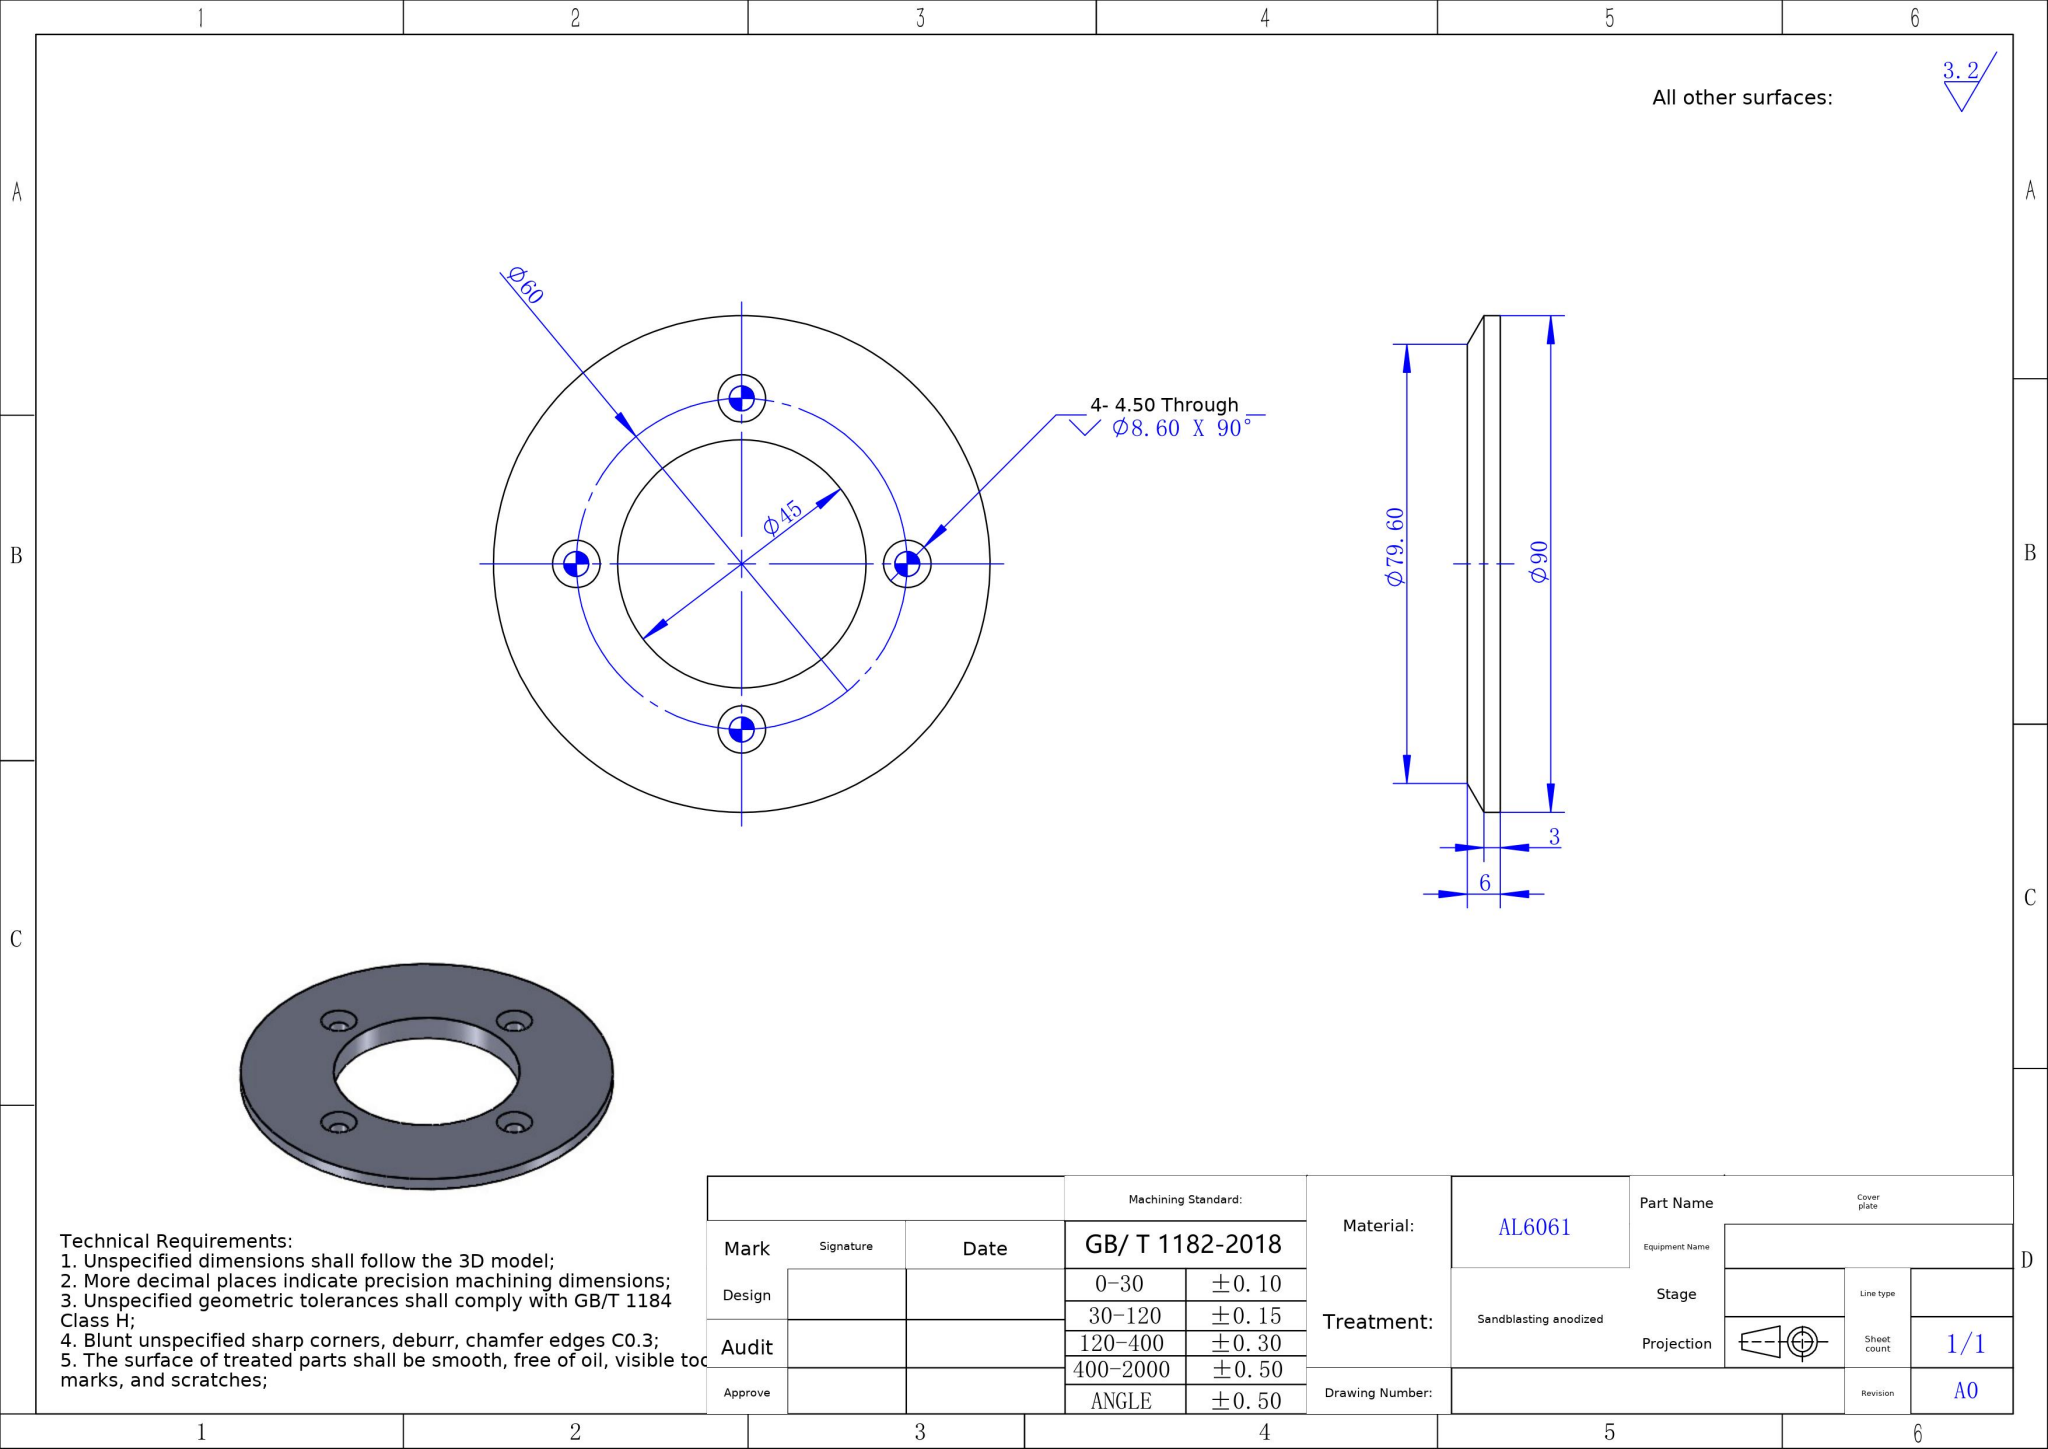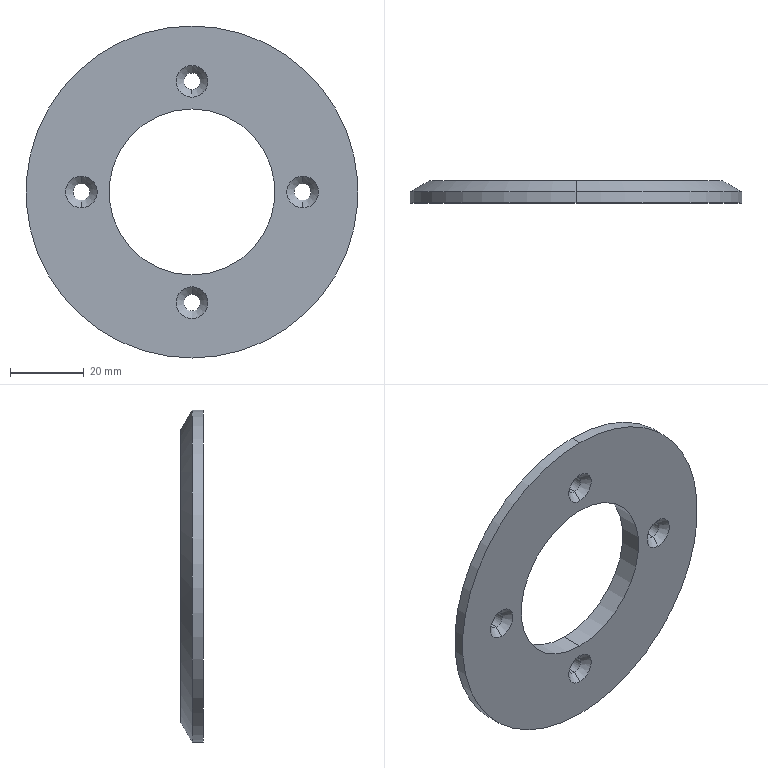Part | SolidWorks | mm | material AL6061 | 1 solid | 24 faces | box 90 x 6 x 90 mm | volume 25971 mm3 | cylinder 12 | cone 10 | plane 2 | commonest cylinder face diameters 4.5 x8 45 x2 90 x2
build123d program:
from build123d import *

# Parameters (mm, degrees)
SKETCH2_R                           = 22.5
CUT_EXTRUDE1_DEPTH                  = 10
SIZE_MM_DOWEL_PIN_HOLE2_D           = 4.5
SIZE_MM_DOWEL_PIN_HOLE2_DEPTH       = 10.7
SIZE_MM_DOWEL_PIN_HOLE2_CSINK_D     = 8.6
SIZE_MM_DOWEL_PIN_HOLE2_CSINK_ANGLE = 90
SIZE_MM_DOWEL_PIN_HOLE2_TIP         = 1.352


with BuildPart() as part:
    # Sketch1 → Revolve1 (revolve)
    with BuildSketch(Plane.XY, mode=Mode.PRIVATE) as revolve1_sk:
        Polygon((0, 0), (45, 0), (45, 3), (39.8, 6), (0, 6), align=None)
    revolve(revolve1_sk.sketch.rotate(Axis((0, 0, 0), (0, 1, 0)), 90), axis=Axis((0, 0, 0), (0, 1, 0)))

    # Sketch2 → Cut-Extrude1 (cut)
    with BuildSketch(Plane.XZ):
        with Locations(Location((0, 0, 0), (0, 0, 270))):
            Circle(SKETCH2_R)
    extrude(amount=-CUT_EXTRUDE1_DEPTH, mode=Mode.SUBTRACT)

    # Size mm Dowel Pin Hole2
    with Locations(Plane(origin=(0, 0, 0), x_dir=(-1, 0, 0), z_dir=(0, -1, 0))):
        with Locations((-30, 0), (0, 30), (30, 0), (0, -30)):
            CounterSinkHole(SIZE_MM_DOWEL_PIN_HOLE2_D / 2, SIZE_MM_DOWEL_PIN_HOLE2_CSINK_D / 2, depth=SIZE_MM_DOWEL_PIN_HOLE2_DEPTH, counter_sink_angle=SIZE_MM_DOWEL_PIN_HOLE2_CSINK_ANGLE)
            with Locations((0, 0, -(SIZE_MM_DOWEL_PIN_HOLE2_DEPTH + SIZE_MM_DOWEL_PIN_HOLE2_TIP / 2))):  # 118° drill point
                Cone(0, SIZE_MM_DOWEL_PIN_HOLE2_D / 2, SIZE_MM_DOWEL_PIN_HOLE2_TIP, mode=Mode.SUBTRACT)


solid = part.part
STEP:
#1=CARTESIAN_POINT('',(0.,2.05,-27.75));
#2=VERTEX_POINT('',#1);
#3=CARTESIAN_POINT('',(0.,2.05,-32.25));
#4=VERTEX_POINT('',#3);
#5=CARTESIAN_POINT('',(0.,2.05,-30.));
#6=DIRECTION('',(0.,-1.,0.));
#7=DIRECTION('',(0.,0.,-1.));
#8=AXIS2_PLACEMENT_3D('',#5,#6,#7);
#9=CIRCLE('',#8,2.25);
#10=EDGE_CURVE('',#2,#4,#9,.T.);
#11=ORIENTED_EDGE('',*,*,#10,.F.);
#12=CARTESIAN_POINT('',(0.,0.,-25.7));
#13=VERTEX_POINT('',#12);
#14=CARTESIAN_POINT('',(0.,0.,-25.7));
#15=DIRECTION('',(0.,-0.7071,0.7071));
#16=VECTOR('',#15,1000.);
#17=LINE('',#14,#16);
#18=EDGE_CURVE('',#2,#13,#17,.T.);
#19=ORIENTED_EDGE('',*,*,#18,.T.);
#20=CARTESIAN_POINT('',(0.,0.,-34.3));
#21=VERTEX_POINT('',#20);
#22=CARTESIAN_POINT('',(0.,0.,-30.));
#23=DIRECTION('',(0.,-1.,0.));
#24=DIRECTION('',(0.,0.,-1.));
#25=AXIS2_PLACEMENT_3D('',#22,#23,#24);
#26=CIRCLE('',#25,4.3);
#27=EDGE_CURVE('',#13,#21,#26,.T.);
#28=ORIENTED_EDGE('',*,*,#27,.T.);
#29=CARTESIAN_POINT('',(0.,0.,-34.3));
#30=DIRECTION('',(0.,-0.7071,-0.7071));
#31=VECTOR('',#30,1000.);
#32=LINE('',#29,#31);
#33=EDGE_CURVE('',#4,#21,#32,.T.);
#34=ORIENTED_EDGE('',*,*,#33,.F.);
#35=EDGE_LOOP('',(#11,#19,#28,#34));
#36=FACE_OUTER_BOUND('',#35,.T.);
#37=CARTESIAN_POINT('',(0.,0.,-30.));
#38=DIRECTION('',(0.,-1.,0.));
#39=DIRECTION('',(0.,0.,-1.));
#40=AXIS2_PLACEMENT_3D('',#37,#38,#39);
#41=CONICAL_SURFACE('',#40,4.3,0.7854);
#42=ADVANCED_FACE('',(#36),#41,.F.);
#43=CARTESIAN_POINT('',(0.,6.,-32.25));
#44=VERTEX_POINT('',#43);
#45=CARTESIAN_POINT('',(0.,6.,-27.75));
#46=VERTEX_POINT('',#45);
#47=CARTESIAN_POINT('',(0.,6.,-30.));
#48=DIRECTION('',(0.,1.,0.));
#49=DIRECTION('',(0.,0.,1.));
#50=AXIS2_PLACEMENT_3D('',#47,#48,#49);
#51=CIRCLE('',#50,2.25);
#52=EDGE_CURVE('',#44,#46,#51,.T.);
#53=ORIENTED_EDGE('',*,*,#52,.T.);
#54=CARTESIAN_POINT('',(0.,0.,-27.75));
#55=DIRECTION('',(0.,-1.,0.));
#56=VECTOR('',#55,1000.);
#57=LINE('',#54,#56);
#58=EDGE_CURVE('',#46,#2,#57,.T.);
#59=ORIENTED_EDGE('',*,*,#58,.T.);
#60=ORIENTED_EDGE('',*,*,#10,.T.);
#61=CARTESIAN_POINT('',(0.,0.,-32.25));
#62=DIRECTION('',(0.,-1.,0.));
#63=VECTOR('',#62,1000.);
#64=LINE('',#61,#63);
#65=EDGE_CURVE('',#44,#4,#64,.T.);
#66=ORIENTED_EDGE('',*,*,#65,.F.);
#67=EDGE_LOOP('',(#53,#59,#60,#66));
#68=FACE_OUTER_BOUND('',#67,.T.);
#69=CARTESIAN_POINT('',(0.,0.,-30.));
#70=DIRECTION('',(0.,-1.,0.));
#71=DIRECTION('',(0.,0.,-1.));
#72=AXIS2_PLACEMENT_3D('',#69,#70,#71);
#73=CYLINDRICAL_SURFACE('',#72,2.25);
#74=ADVANCED_FACE('',(#68),#73,.F.);
#75=CARTESIAN_POINT('',(-30.,2.05,2.25));
#76=VERTEX_POINT('',#75);
#77=CARTESIAN_POINT('',(-30.,2.05,-2.25));
#78=VERTEX_POINT('',#77);
#79=CARTESIAN_POINT('',(-30.,2.05,-0.));
#80=DIRECTION('',(0.,-1.,0.));
#81=DIRECTION('',(0.,0.,-1.));
#82=AXIS2_PLACEMENT_3D('',#79,#80,#81);
#83=CIRCLE('',#82,2.25);
#84=EDGE_CURVE('',#76,#78,#83,.T.);
#85=ORIENTED_EDGE('',*,*,#84,.F.);
#86=CARTESIAN_POINT('',(-30.,0.,4.3));
#87=VERTEX_POINT('',#86);
#88=CARTESIAN_POINT('',(-30.,0.,4.3));
#89=DIRECTION('',(0.,-0.7071,0.7071));
#90=VECTOR('',#89,1000.);
#91=LINE('',#88,#90);
#92=EDGE_CURVE('',#76,#87,#91,.T.);
#93=ORIENTED_EDGE('',*,*,#92,.T.);
#94=CARTESIAN_POINT('',(-30.,0.,-4.3));
#95=VERTEX_POINT('',#94);
#96=CARTESIAN_POINT('',(-30.,0.,-0.));
#97=DIRECTION('',(0.,-1.,0.));
#98=DIRECTION('',(0.,0.,-1.));
#99=AXIS2_PLACEMENT_3D('',#96,#97,#98);
#100=CIRCLE('',#99,4.3);
#101=EDGE_CURVE('',#87,#95,#100,.T.);
#102=ORIENTED_EDGE('',*,*,#101,.T.);
#103=CARTESIAN_POINT('',(-30.,0.,-4.3));
#104=DIRECTION('',(0.,-0.7071,-0.7071));
#105=VECTOR('',#104,1000.);
#106=LINE('',#103,#105);
#107=EDGE_CURVE('',#78,#95,#106,.T.);
#108=ORIENTED_EDGE('',*,*,#107,.F.);
#109=EDGE_LOOP('',(#85,#93,#102,#108));
#110=FACE_OUTER_BOUND('',#109,.T.);
#111=CARTESIAN_POINT('',(-30.,0.,-0.));
#112=DIRECTION('',(0.,-1.,0.));
#113=DIRECTION('',(0.,0.,-1.));
#114=AXIS2_PLACEMENT_3D('',#111,#112,#113);
#115=CONICAL_SURFACE('',#114,4.3,0.7854);
#116=ADVANCED_FACE('',(#110),#115,.F.);
#117=CARTESIAN_POINT('',(-30.,6.,-2.25));
#118=VERTEX_POINT('',#117);
#119=CARTESIAN_POINT('',(-30.,6.,2.25));
#120=VERTEX_POINT('',#119);
#121=CARTESIAN_POINT('',(-30.,6.,-0.));
#122=DIRECTION('',(0.,1.,0.));
#123=DIRECTION('',(0.,0.,1.));
#124=AXIS2_PLACEMENT_3D('',#121,#122,#123);
#125=CIRCLE('',#124,2.25);
#126=EDGE_CURVE('',#118,#120,#125,.T.);
#127=ORIENTED_EDGE('',*,*,#126,.T.);
#128=CARTESIAN_POINT('',(-30.,0.,2.25));
#129=DIRECTION('',(0.,-1.,0.));
#130=VECTOR('',#129,1000.);
#131=LINE('',#128,#130);
#132=EDGE_CURVE('',#120,#76,#131,.T.);
#133=ORIENTED_EDGE('',*,*,#132,.T.);
#134=ORIENTED_EDGE('',*,*,#84,.T.);
#135=CARTESIAN_POINT('',(-30.,0.,-2.25));
#136=DIRECTION('',(0.,-1.,0.));
#137=VECTOR('',#136,1000.);
#138=LINE('',#135,#137);
#139=EDGE_CURVE('',#118,#78,#138,.T.);
#140=ORIENTED_EDGE('',*,*,#139,.F.);
#141=EDGE_LOOP('',(#127,#133,#134,#140));
#142=FACE_OUTER_BOUND('',#141,.T.);
#143=CARTESIAN_POINT('',(-30.,0.,-0.));
#144=DIRECTION('',(0.,-1.,0.));
#145=DIRECTION('',(0.,0.,-1.));
#146=AXIS2_PLACEMENT_3D('',#143,#144,#145);
#147=CYLINDRICAL_SURFACE('',#146,2.25);
#148=ADVANCED_FACE('',(#142),#147,.F.);
#149=CARTESIAN_POINT('',(-0.,2.05,32.25));
#150=VERTEX_POINT('',#149);
#151=CARTESIAN_POINT('',(-0.,2.05,27.75));
#152=VERTEX_POINT('',#151);
#153=CARTESIAN_POINT('',(-0.,2.05,30.));
#154=DIRECTION('',(0.,-1.,0.));
#155=DIRECTION('',(0.,0.,-1.));
#156=AXIS2_PLACEMENT_3D('',#153,#154,#155);
#157=CIRCLE('',#156,2.25);
#158=EDGE_CURVE('',#150,#152,#157,.T.);
#159=ORIENTED_EDGE('',*,*,#158,.F.);
#160=CARTESIAN_POINT('',(-0.,0.,34.3));
#161=VERTEX_POINT('',#160);
#162=CARTESIAN_POINT('',(-0.,0.,34.3));
#163=DIRECTION('',(0.,-0.7071,0.7071));
#164=VECTOR('',#163,1000.);
#165=LINE('',#162,#164);
#166=EDGE_CURVE('',#150,#161,#165,.T.);
#167=ORIENTED_EDGE('',*,*,#166,.T.);
#168=CARTESIAN_POINT('',(-0.,0.,25.7));
#169=VERTEX_POINT('',#168);
#170=CARTESIAN_POINT('',(-0.,0.,30.));
#171=DIRECTION('',(0.,-1.,0.));
#172=DIRECTION('',(0.,0.,-1.));
#173=AXIS2_PLACEMENT_3D('',#170,#171,#172);
#174=CIRCLE('',#173,4.3);
#175=EDGE_CURVE('',#161,#169,#174,.T.);
#176=ORIENTED_EDGE('',*,*,#175,.T.);
#177=CARTESIAN_POINT('',(-0.,0.,25.7));
#178=DIRECTION('',(0.,-0.7071,-0.7071));
#179=VECTOR('',#178,1000.);
#180=LINE('',#177,#179);
#181=EDGE_CURVE('',#152,#169,#180,.T.);
#182=ORIENTED_EDGE('',*,*,#181,.F.);
#183=EDGE_LOOP('',(#159,#167,#176,#182));
#184=FACE_OUTER_BOUND('',#183,.T.);
#185=CARTESIAN_POINT('',(-0.,0.,30.));
#186=DIRECTION('',(0.,-1.,0.));
#187=DIRECTION('',(0.,0.,-1.));
#188=AXIS2_PLACEMENT_3D('',#185,#186,#187);
#189=CONICAL_SURFACE('',#188,4.3,0.7854);
#190=ADVANCED_FACE('',(#184),#189,.F.);
#191=CARTESIAN_POINT('',(-0.,6.,27.75));
#192=VERTEX_POINT('',#191);
#193=CARTESIAN_POINT('',(-0.,6.,32.25));
#194=VERTEX_POINT('',#193);
#195=CARTESIAN_POINT('',(-0.,6.,30.));
#196=DIRECTION('',(0.,1.,0.));
#197=DIRECTION('',(0.,0.,1.));
#198=AXIS2_PLACEMENT_3D('',#195,#196,#197);
#199=CIRCLE('',#198,2.25);
#200=EDGE_CURVE('',#192,#194,#199,.T.);
#201=ORIENTED_EDGE('',*,*,#200,.T.);
#202=CARTESIAN_POINT('',(-0.,0.,32.25));
#203=DIRECTION('',(0.,-1.,0.));
#204=VECTOR('',#203,1000.);
#205=LINE('',#202,#204);
#206=EDGE_CURVE('',#194,#150,#205,.T.);
#207=ORIENTED_EDGE('',*,*,#206,.T.);
#208=ORIENTED_EDGE('',*,*,#158,.T.);
#209=CARTESIAN_POINT('',(-0.,0.,27.75));
#210=DIRECTION('',(0.,-1.,0.));
#211=VECTOR('',#210,1000.);
#212=LINE('',#209,#211);
#213=EDGE_CURVE('',#192,#152,#212,.T.);
#214=ORIENTED_EDGE('',*,*,#213,.F.);
#215=EDGE_LOOP('',(#201,#207,#208,#214));
#216=FACE_OUTER_BOUND('',#215,.T.);
#217=CARTESIAN_POINT('',(-0.,0.,30.));
#218=DIRECTION('',(0.,-1.,0.));
#219=DIRECTION('',(0.,0.,-1.));
#220=AXIS2_PLACEMENT_3D('',#217,#218,#219);
#221=CYLINDRICAL_SURFACE('',#220,2.25);
#222=ADVANCED_FACE('',(#216),#221,.F.);
#223=CARTESIAN_POINT('',(30.,2.05,2.25));
#224=VERTEX_POINT('',#223);
#225=CARTESIAN_POINT('',(30.,2.05,-2.25));
#226=VERTEX_POINT('',#225);
#227=CARTESIAN_POINT('',(30.,2.05,0.));
#228=DIRECTION('',(0.,-1.,0.));
#229=DIRECTION('',(0.,0.,-1.));
#230=AXIS2_PLACEMENT_3D('',#227,#228,#229);
#231=CIRCLE('',#230,2.25);
#232=EDGE_CURVE('',#224,#226,#231,.T.);
#233=ORIENTED_EDGE('',*,*,#232,.F.);
#234=CARTESIAN_POINT('',(30.,0.,4.3));
#235=VERTEX_POINT('',#234);
#236=CARTESIAN_POINT('',(30.,0.,4.3));
#237=DIRECTION('',(0.,-0.7071,0.7071));
#238=VECTOR('',#237,1000.);
#239=LINE('',#236,#238);
#240=EDGE_CURVE('',#224,#235,#239,.T.);
#241=ORIENTED_EDGE('',*,*,#240,.T.);
#242=CARTESIAN_POINT('',(30.,0.,-4.3));
#243=VERTEX_POINT('',#242);
#244=CARTESIAN_POINT('',(30.,0.,0.));
#245=DIRECTION('',(0.,-1.,0.));
#246=DIRECTION('',(0.,0.,-1.));
#247=AXIS2_PLACEMENT_3D('',#244,#245,#246);
#248=CIRCLE('',#247,4.3);
#249=EDGE_CURVE('',#235,#243,#248,.T.);
#250=ORIENTED_EDGE('',*,*,#249,.T.);
#251=CARTESIAN_POINT('',(30.,0.,-4.3));
#252=DIRECTION('',(0.,-0.7071,-0.7071));
#253=VECTOR('',#252,1000.);
#254=LINE('',#251,#253);
#255=EDGE_CURVE('',#226,#243,#254,.T.);
#256=ORIENTED_EDGE('',*,*,#255,.F.);
#257=EDGE_LOOP('',(#233,#241,#250,#256));
#258=FACE_OUTER_BOUND('',#257,.T.);
#259=CARTESIAN_POINT('',(30.,0.,0.));
#260=DIRECTION('',(0.,-1.,0.));
#261=DIRECTION('',(0.,0.,-1.));
#262=AXIS2_PLACEMENT_3D('',#259,#260,#261);
#263=CONICAL_SURFACE('',#262,4.3,0.7854);
#264=ADVANCED_FACE('',(#258),#263,.F.);
#265=CARTESIAN_POINT('',(30.,6.,-2.25));
#266=VERTEX_POINT('',#265);
#267=CARTESIAN_POINT('',(30.,6.,2.25));
#268=VERTEX_POINT('',#267);
#269=CARTESIAN_POINT('',(30.,6.,0.));
#270=DIRECTION('',(0.,1.,0.));
#271=DIRECTION('',(0.,0.,1.));
#272=AXIS2_PLACEMENT_3D('',#269,#270,#271);
#273=CIRCLE('',#272,2.25);
#274=EDGE_CURVE('',#266,#268,#273,.T.);
#275=ORIENTED_EDGE('',*,*,#274,.T.);
#276=CARTESIAN_POINT('',(30.,0.,2.25));
#277=DIRECTION('',(0.,-1.,0.));
#278=VECTOR('',#277,1000.);
#279=LINE('',#276,#278);
#280=EDGE_CURVE('',#268,#224,#279,.T.);
#281=ORIENTED_EDGE('',*,*,#280,.T.);
#282=ORIENTED_EDGE('',*,*,#232,.T.);
#283=CARTESIAN_POINT('',(30.,0.,-2.25));
#284=DIRECTION('',(0.,-1.,0.));
#285=VECTOR('',#284,1000.);
#286=LINE('',#283,#285);
#287=EDGE_CURVE('',#266,#226,#286,.T.);
#288=ORIENTED_EDGE('',*,*,#287,.F.);
#289=EDGE_LOOP('',(#275,#281,#282,#288));
#290=FACE_OUTER_BOUND('',#289,.T.);
#291=CARTESIAN_POINT('',(30.,0.,0.));
#292=DIRECTION('',(0.,-1.,0.));
#293=DIRECTION('',(0.,0.,-1.));
#294=AXIS2_PLACEMENT_3D('',#291,#292,#293);
#295=CYLINDRICAL_SURFACE('',#294,2.25);
#296=ADVANCED_FACE('',(#290),#295,.F.);
#297=CARTESIAN_POINT('',(0.,6.,-22.5));
#298=VERTEX_POINT('',#297);
#299=CARTESIAN_POINT('',(0.,6.,22.5));
#300=VERTEX_POINT('',#299);
#301=CARTESIAN_POINT('',(0.,6.,0.));
#302=DIRECTION('',(0.,1.,0.));
#303=DIRECTION('',(0.,0.,1.));
#304=AXIS2_PLACEMENT_3D('',#301,#302,#303);
#305=CIRCLE('',#304,22.5);
#306=EDGE_CURVE('',#298,#300,#305,.T.);
#307=ORIENTED_EDGE('',*,*,#306,.T.);
#308=CARTESIAN_POINT('',(0.,0.,22.5));
#309=VERTEX_POINT('',#308);
#310=CARTESIAN_POINT('',(0.,10.,22.5));
#311=DIRECTION('',(0.,-1.,0.));
#312=VECTOR('',#311,1000.);
#313=LINE('',#310,#312);
#314=EDGE_CURVE('',#300,#309,#313,.T.);
#315=ORIENTED_EDGE('',*,*,#314,.T.);
#316=CARTESIAN_POINT('',(0.,0.,-22.5));
#317=VERTEX_POINT('',#316);
#318=CARTESIAN_POINT('',(0.,0.,0.));
#319=DIRECTION('',(0.,-1.,0.));
#320=DIRECTION('',(0.,0.,-1.));
#321=AXIS2_PLACEMENT_3D('',#318,#319,#320);
#322=CIRCLE('',#321,22.5);
#323=EDGE_CURVE('',#309,#317,#322,.T.);
#324=ORIENTED_EDGE('',*,*,#323,.T.);
#325=CARTESIAN_POINT('',(0.,10.,-22.5));
#326=DIRECTION('',(0.,-1.,0.));
#327=VECTOR('',#326,1000.);
#328=LINE('',#325,#327);
#329=EDGE_CURVE('',#298,#317,#328,.T.);
#330=ORIENTED_EDGE('',*,*,#329,.F.);
#331=EDGE_LOOP('',(#307,#315,#324,#330));
#332=FACE_OUTER_BOUND('',#331,.T.);
#333=CARTESIAN_POINT('',(0.,10.,0.));
#334=DIRECTION('',(0.,-1.,0.));
#335=DIRECTION('',(0.,0.,-1.));
#336=AXIS2_PLACEMENT_3D('',#333,#334,#335);
#337=CYLINDRICAL_SURFACE('',#336,22.5);
#338=ADVANCED_FACE('',(#332),#337,.F.);
#339=CARTESIAN_POINT('',(0.,6.,-39.8));
#340=VERTEX_POINT('',#339);
#341=CARTESIAN_POINT('',(0.,6.,39.8));
#342=VERTEX_POINT('',#341);
#343=CARTESIAN_POINT('',(0.,6.,0.));
#344=DIRECTION('',(0.,-1.,0.));
#345=DIRECTION('',(0.,0.,-1.));
#346=AXIS2_PLACEMENT_3D('',#343,#344,#345);
#347=CIRCLE('',#346,39.8);
#348=EDGE_CURVE('',#340,#342,#347,.T.);
#349=ORIENTED_EDGE('',*,*,#348,.T.);
#350=CARTESIAN_POINT('',(0.,3.,45.));
#351=VERTEX_POINT('',#350);
#352=CARTESIAN_POINT('',(0.,3.,45.));
#353=DIRECTION('',(0.,-0.4997,0.8662));
#354=VECTOR('',#353,1000.);
#355=LINE('',#352,#354);
#356=EDGE_CURVE('',#342,#351,#355,.T.);
#357=ORIENTED_EDGE('',*,*,#356,.T.);
#358=CARTESIAN_POINT('',(0.,3.,-45.));
#359=VERTEX_POINT('',#358);
#360=CARTESIAN_POINT('',(0.,3.,0.));
#361=DIRECTION('',(0.,-1.,0.));
#362=DIRECTION('',(0.,0.,-1.));
#363=AXIS2_PLACEMENT_3D('',#360,#361,#362);
#364=CIRCLE('',#363,45.);
#365=EDGE_CURVE('',#359,#351,#364,.T.);
#366=ORIENTED_EDGE('',*,*,#365,.F.);
#367=CARTESIAN_POINT('',(0.,3.,-45.));
#368=DIRECTION('',(0.,-0.4997,-0.8662));
#369=VECTOR('',#368,1000.);
#370=LINE('',#367,#369);
#371=EDGE_CURVE('',#340,#359,#370,.T.);
#372=ORIENTED_EDGE('',*,*,#371,.F.);
#373=EDGE_LOOP('',(#349,#357,#366,#372));
#374=FACE_OUTER_BOUND('',#373,.T.);
#375=CARTESIAN_POINT('',(0.,3.,0.));
#376=DIRECTION('',(0.,-1.,0.));
#377=DIRECTION('',(0.,0.,-1.));
#378=AXIS2_PLACEMENT_3D('',#375,#376,#377);
#379=CONICAL_SURFACE('',#378,45.,1.048);
#380=ADVANCED_FACE('',(#374),#379,.T.);
#381=ORIENTED_EDGE('',*,*,#365,.T.);
#382=CARTESIAN_POINT('',(0.,0.,45.));
#383=VERTEX_POINT('',#382);
#384=CARTESIAN_POINT('',(0.,0.,45.));
#385=DIRECTION('',(0.,-1.,0.));
#386=VECTOR('',#385,1000.);
#387=LINE('',#384,#386);
#388=EDGE_CURVE('',#351,#383,#387,.T.);
#389=ORIENTED_EDGE('',*,*,#388,.T.);
#390=CARTESIAN_POINT('',(0.,0.,-45.));
#391=VERTEX_POINT('',#390);
#392=CARTESIAN_POINT('',(0.,0.,0.));
#393=DIRECTION('',(0.,-1.,0.));
#394=DIRECTION('',(0.,0.,-1.));
#395=AXIS2_PLACEMENT_3D('',#392,#393,#394);
#396=CIRCLE('',#395,45.);
#397=EDGE_CURVE('',#391,#383,#396,.T.);
#398=ORIENTED_EDGE('',*,*,#397,.F.);
#399=CARTESIAN_POINT('',(0.,0.,-45.));
#400=DIRECTION('',(0.,-1.,0.));
#401=VECTOR('',#400,1000.);
#402=LINE('',#399,#401);
#403=EDGE_CURVE('',#359,#391,#402,.T.);
#404=ORIENTED_EDGE('',*,*,#403,.F.);
#405=EDGE_LOOP('',(#381,#389,#398,#404));
#406=FACE_OUTER_BOUND('',#405,.T.);
#407=CARTESIAN_POINT('',(0.,0.,0.));
#408=DIRECTION('',(0.,-1.,0.));
#409=DIRECTION('',(0.,0.,-1.));
#410=AXIS2_PLACEMENT_3D('',#407,#408,#409);
#411=CYLINDRICAL_SURFACE('',#410,45.);
#412=ADVANCED_FACE('',(#406),#411,.T.);
#413=CARTESIAN_POINT('',(0.,0.,-30.));
#414=DIRECTION('',(0.,-1.,0.));
#415=DIRECTION('',(0.,0.,-1.));
#416=AXIS2_PLACEMENT_3D('',#413,#414,#415);
#417=CIRCLE('',#416,4.3);
#418=EDGE_CURVE('',#21,#13,#417,.T.);
#419=ORIENTED_EDGE('',*,*,#418,.F.);
#420=ORIENTED_EDGE('',*,*,#27,.F.);
#421=EDGE_LOOP('',(#419,#420));
#422=FACE_BOUND('',#421,.T.);
#423=CARTESIAN_POINT('',(-30.,0.,-0.));
#424=DIRECTION('',(0.,-1.,0.));
#425=DIRECTION('',(0.,0.,-1.));
#426=AXIS2_PLACEMENT_3D('',#423,#424,#425);
#427=CIRCLE('',#426,4.3);
#428=EDGE_CURVE('',#95,#87,#427,.T.);
#429=ORIENTED_EDGE('',*,*,#428,.F.);
#430=ORIENTED_EDGE('',*,*,#101,.F.);
#431=EDGE_LOOP('',(#429,#430));
#432=FACE_BOUND('',#431,.T.);
#433=CARTESIAN_POINT('',(-0.,0.,30.));
#434=DIRECTION('',(0.,-1.,0.));
#435=DIRECTION('',(0.,0.,-1.));
#436=AXIS2_PLACEMENT_3D('',#433,#434,#435);
#437=CIRCLE('',#436,4.3);
#438=EDGE_CURVE('',#169,#161,#437,.T.);
#439=ORIENTED_EDGE('',*,*,#438,.F.);
#440=ORIENTED_EDGE('',*,*,#175,.F.);
#441=EDGE_LOOP('',(#439,#440));
#442=FACE_BOUND('',#441,.T.);
#443=CARTESIAN_POINT('',(30.,0.,0.));
#444=DIRECTION('',(0.,-1.,0.));
#445=DIRECTION('',(0.,0.,-1.));
#446=AXIS2_PLACEMENT_3D('',#443,#444,#445);
#447=CIRCLE('',#446,4.3);
#448=EDGE_CURVE('',#243,#235,#447,.T.);
#449=ORIENTED_EDGE('',*,*,#448,.F.);
#450=ORIENTED_EDGE('',*,*,#249,.F.);
#451=EDGE_LOOP('',(#449,#450));
#452=FACE_BOUND('',#451,.T.);
#453=CARTESIAN_POINT('',(0.,0.,0.));
#454=DIRECTION('',(0.,-1.,0.));
#455=DIRECTION('',(0.,0.,-1.));
#456=AXIS2_PLACEMENT_3D('',#453,#454,#455);
#457=CIRCLE('',#456,22.5);
#458=EDGE_CURVE('',#317,#309,#457,.T.);
#459=ORIENTED_EDGE('',*,*,#458,.F.);
#460=ORIENTED_EDGE('',*,*,#323,.F.);
#461=EDGE_LOOP('',(#459,#460));
#462=FACE_BOUND('',#461,.T.);
#463=ORIENTED_EDGE('',*,*,#397,.T.);
#464=CARTESIAN_POINT('',(0.,0.,0.));
#465=DIRECTION('',(0.,-1.,0.));
#466=DIRECTION('',(0.,0.,-1.));
#467=AXIS2_PLACEMENT_3D('',#464,#465,#466);
#468=CIRCLE('',#467,45.);
#469=EDGE_CURVE('',#383,#391,#468,.T.);
#470=ORIENTED_EDGE('',*,*,#469,.T.);
#471=EDGE_LOOP('',(#463,#470));
#472=FACE_OUTER_BOUND('',#471,.T.);
#473=CARTESIAN_POINT('',(0.,0.,0.));
#474=DIRECTION('',(0.,-1.,0.));
#475=DIRECTION('',(0.,0.,-1.));
#476=AXIS2_PLACEMENT_3D('',#473,#474,#475);
#477=PLANE('',#476);
#478=ADVANCED_FACE('',(#422,#432,#442,#452,#462,#472),#477,.T.);
#479=ORIENTED_EDGE('',*,*,#388,.F.);
#480=CARTESIAN_POINT('',(0.,3.,0.));
#481=DIRECTION('',(0.,-1.,0.));
#482=DIRECTION('',(0.,0.,-1.));
#483=AXIS2_PLACEMENT_3D('',#480,#481,#482);
#484=CIRCLE('',#483,45.);
#485=EDGE_CURVE('',#351,#359,#484,.T.);
#486=ORIENTED_EDGE('',*,*,#485,.T.);
#487=ORIENTED_EDGE('',*,*,#403,.T.);
#488=ORIENTED_EDGE('',*,*,#469,.F.);
#489=EDGE_LOOP('',(#479,#486,#487,#488));
#490=FACE_OUTER_BOUND('',#489,.T.);
#491=CARTESIAN_POINT('',(0.,0.,0.));
#492=DIRECTION('',(0.,-1.,0.));
#493=DIRECTION('',(0.,0.,-1.));
#494=AXIS2_PLACEMENT_3D('',#491,#492,#493);
#495=CYLINDRICAL_SURFACE('',#494,45.);
#496=ADVANCED_FACE('',(#490),#495,.T.);
#497=ORIENTED_EDGE('',*,*,#356,.F.);
#498=CARTESIAN_POINT('',(0.,6.,0.));
#499=DIRECTION('',(0.,-1.,0.));
#500=DIRECTION('',(0.,0.,-1.));
#501=AXIS2_PLACEMENT_3D('',#498,#499,#500);
#502=CIRCLE('',#501,39.8);
#503=EDGE_CURVE('',#342,#340,#502,.T.);
#504=ORIENTED_EDGE('',*,*,#503,.T.);
#505=ORIENTED_EDGE('',*,*,#371,.T.);
#506=ORIENTED_EDGE('',*,*,#485,.F.);
#507=EDGE_LOOP('',(#497,#504,#505,#506));
#508=FACE_OUTER_BOUND('',#507,.T.);
#509=CARTESIAN_POINT('',(0.,3.,0.));
#510=DIRECTION('',(0.,-1.,0.));
#511=DIRECTION('',(0.,0.,-1.));
#512=AXIS2_PLACEMENT_3D('',#509,#510,#511);
#513=CONICAL_SURFACE('',#512,45.,1.048);
#514=ADVANCED_FACE('',(#508),#513,.T.);
#515=ORIENTED_EDGE('',*,*,#52,.F.);
#516=CARTESIAN_POINT('',(0.,6.,-30.));
#517=DIRECTION('',(0.,1.,0.));
#518=DIRECTION('',(0.,0.,1.));
#519=AXIS2_PLACEMENT_3D('',#516,#517,#518);
#520=CIRCLE('',#519,2.25);
#521=EDGE_CURVE('',#46,#44,#520,.T.);
#522=ORIENTED_EDGE('',*,*,#521,.F.);
#523=EDGE_LOOP('',(#515,#522));
#524=FACE_BOUND('',#523,.T.);
#525=ORIENTED_EDGE('',*,*,#126,.F.);
#526=CARTESIAN_POINT('',(-30.,6.,-0.));
#527=DIRECTION('',(0.,1.,0.));
#528=DIRECTION('',(0.,0.,1.));
#529=AXIS2_PLACEMENT_3D('',#526,#527,#528);
#530=CIRCLE('',#529,2.25);
#531=EDGE_CURVE('',#120,#118,#530,.T.);
#532=ORIENTED_EDGE('',*,*,#531,.F.);
#533=EDGE_LOOP('',(#525,#532));
#534=FACE_BOUND('',#533,.T.);
#535=ORIENTED_EDGE('',*,*,#200,.F.);
#536=CARTESIAN_POINT('',(-0.,6.,30.));
#537=DIRECTION('',(0.,1.,0.));
#538=DIRECTION('',(0.,0.,1.));
#539=AXIS2_PLACEMENT_3D('',#536,#537,#538);
#540=CIRCLE('',#539,2.25);
#541=EDGE_CURVE('',#194,#192,#540,.T.);
#542=ORIENTED_EDGE('',*,*,#541,.F.);
#543=EDGE_LOOP('',(#535,#542));
#544=FACE_BOUND('',#543,.T.);
#545=ORIENTED_EDGE('',*,*,#274,.F.);
#546=CARTESIAN_POINT('',(30.,6.,0.));
#547=DIRECTION('',(0.,1.,0.));
#548=DIRECTION('',(0.,0.,1.));
#549=AXIS2_PLACEMENT_3D('',#546,#547,#548);
#550=CIRCLE('',#549,2.25);
#551=EDGE_CURVE('',#268,#266,#550,.T.);
#552=ORIENTED_EDGE('',*,*,#551,.F.);
#553=EDGE_LOOP('',(#545,#552));
#554=FACE_BOUND('',#553,.T.);
#555=ORIENTED_EDGE('',*,*,#306,.F.);
#556=CARTESIAN_POINT('',(0.,6.,0.));
#557=DIRECTION('',(0.,1.,0.));
#558=DIRECTION('',(0.,0.,1.));
#559=AXIS2_PLACEMENT_3D('',#556,#557,#558);
#560=CIRCLE('',#559,22.5);
#561=EDGE_CURVE('',#300,#298,#560,.T.);
#562=ORIENTED_EDGE('',*,*,#561,.F.);
#563=EDGE_LOOP('',(#555,#562));
#564=FACE_BOUND('',#563,.T.);
#565=ORIENTED_EDGE('',*,*,#348,.F.);
#566=ORIENTED_EDGE('',*,*,#503,.F.);
#567=EDGE_LOOP('',(#565,#566));
#568=FACE_OUTER_BOUND('',#567,.T.);
#569=CARTESIAN_POINT('',(39.8,6.,0.));
#570=DIRECTION('',(0.,1.,0.));
#571=DIRECTION('',(0.,0.,1.));
#572=AXIS2_PLACEMENT_3D('',#569,#570,#571);
#573=PLANE('',#572);
#574=ADVANCED_FACE('',(#524,#534,#544,#554,#564,#568),#573,.T.);
#575=ORIENTED_EDGE('',*,*,#314,.F.);
#576=ORIENTED_EDGE('',*,*,#561,.T.);
#577=ORIENTED_EDGE('',*,*,#329,.T.);
#578=ORIENTED_EDGE('',*,*,#458,.T.);
#579=EDGE_LOOP('',(#575,#576,#577,#578));
#580=FACE_OUTER_BOUND('',#579,.T.);
#581=CARTESIAN_POINT('',(0.,10.,0.));
#582=DIRECTION('',(0.,-1.,0.));
#583=DIRECTION('',(0.,0.,-1.));
#584=AXIS2_PLACEMENT_3D('',#581,#582,#583);
#585=CYLINDRICAL_SURFACE('',#584,22.5);
#586=ADVANCED_FACE('',(#580),#585,.F.);
#587=ORIENTED_EDGE('',*,*,#280,.F.);
#588=ORIENTED_EDGE('',*,*,#551,.T.);
#589=ORIENTED_EDGE('',*,*,#287,.T.);
#590=CARTESIAN_POINT('',(30.,2.05,0.));
#591=DIRECTION('',(0.,-1.,0.));
#592=DIRECTION('',(0.,0.,-1.));
#593=AXIS2_PLACEMENT_3D('',#590,#591,#592);
#594=CIRCLE('',#593,2.25);
#595=EDGE_CURVE('',#226,#224,#594,.T.);
#596=ORIENTED_EDGE('',*,*,#595,.T.);
#597=EDGE_LOOP('',(#587,#588,#589,#596));
#598=FACE_OUTER_BOUND('',#597,.T.);
#599=CARTESIAN_POINT('',(30.,0.,0.));
#600=DIRECTION('',(0.,-1.,0.));
#601=DIRECTION('',(0.,0.,-1.));
#602=AXIS2_PLACEMENT_3D('',#599,#600,#601);
#603=CYLINDRICAL_SURFACE('',#602,2.25);
#604=ADVANCED_FACE('',(#598),#603,.F.);
#605=ORIENTED_EDGE('',*,*,#240,.F.);
#606=ORIENTED_EDGE('',*,*,#595,.F.);
#607=ORIENTED_EDGE('',*,*,#255,.T.);
#608=ORIENTED_EDGE('',*,*,#448,.T.);
#609=EDGE_LOOP('',(#605,#606,#607,#608));
#610=FACE_OUTER_BOUND('',#609,.T.);
#611=CARTESIAN_POINT('',(30.,0.,0.));
#612=DIRECTION('',(0.,-1.,0.));
#613=DIRECTION('',(0.,0.,-1.));
#614=AXIS2_PLACEMENT_3D('',#611,#612,#613);
#615=CONICAL_SURFACE('',#614,4.3,0.7854);
#616=ADVANCED_FACE('',(#610),#615,.F.);
#617=ORIENTED_EDGE('',*,*,#206,.F.);
#618=ORIENTED_EDGE('',*,*,#541,.T.);
#619=ORIENTED_EDGE('',*,*,#213,.T.);
#620=CARTESIAN_POINT('',(-0.,2.05,30.));
#621=DIRECTION('',(0.,-1.,0.));
#622=DIRECTION('',(0.,0.,-1.));
#623=AXIS2_PLACEMENT_3D('',#620,#621,#622);
#624=CIRCLE('',#623,2.25);
#625=EDGE_CURVE('',#152,#150,#624,.T.);
#626=ORIENTED_EDGE('',*,*,#625,.T.);
#627=EDGE_LOOP('',(#617,#618,#619,#626));
#628=FACE_OUTER_BOUND('',#627,.T.);
#629=CARTESIAN_POINT('',(-0.,0.,30.));
#630=DIRECTION('',(0.,-1.,0.));
#631=DIRECTION('',(0.,0.,-1.));
#632=AXIS2_PLACEMENT_3D('',#629,#630,#631);
#633=CYLINDRICAL_SURFACE('',#632,2.25);
#634=ADVANCED_FACE('',(#628),#633,.F.);
#635=ORIENTED_EDGE('',*,*,#166,.F.);
#636=ORIENTED_EDGE('',*,*,#625,.F.);
#637=ORIENTED_EDGE('',*,*,#181,.T.);
#638=ORIENTED_EDGE('',*,*,#438,.T.);
#639=EDGE_LOOP('',(#635,#636,#637,#638));
#640=FACE_OUTER_BOUND('',#639,.T.);
#641=CARTESIAN_POINT('',(-0.,0.,30.));
#642=DIRECTION('',(0.,-1.,0.));
#643=DIRECTION('',(0.,0.,-1.));
#644=AXIS2_PLACEMENT_3D('',#641,#642,#643);
#645=CONICAL_SURFACE('',#644,4.3,0.7854);
#646=ADVANCED_FACE('',(#640),#645,.F.);
#647=ORIENTED_EDGE('',*,*,#132,.F.);
#648=ORIENTED_EDGE('',*,*,#531,.T.);
#649=ORIENTED_EDGE('',*,*,#139,.T.);
#650=CARTESIAN_POINT('',(-30.,2.05,-0.));
#651=DIRECTION('',(0.,-1.,0.));
#652=DIRECTION('',(0.,0.,-1.));
#653=AXIS2_PLACEMENT_3D('',#650,#651,#652);
#654=CIRCLE('',#653,2.25);
#655=EDGE_CURVE('',#78,#76,#654,.T.);
#656=ORIENTED_EDGE('',*,*,#655,.T.);
#657=EDGE_LOOP('',(#647,#648,#649,#656));
#658=FACE_OUTER_BOUND('',#657,.T.);
#659=CARTESIAN_POINT('',(-30.,0.,-0.));
#660=DIRECTION('',(0.,-1.,0.));
#661=DIRECTION('',(0.,0.,-1.));
#662=AXIS2_PLACEMENT_3D('',#659,#660,#661);
#663=CYLINDRICAL_SURFACE('',#662,2.25);
#664=ADVANCED_FACE('',(#658),#663,.F.);
#665=ORIENTED_EDGE('',*,*,#92,.F.);
#666=ORIENTED_EDGE('',*,*,#655,.F.);
#667=ORIENTED_EDGE('',*,*,#107,.T.);
#668=ORIENTED_EDGE('',*,*,#428,.T.);
#669=EDGE_LOOP('',(#665,#666,#667,#668));
#670=FACE_OUTER_BOUND('',#669,.T.);
#671=CARTESIAN_POINT('',(-30.,0.,-0.));
#672=DIRECTION('',(0.,-1.,0.));
#673=DIRECTION('',(0.,0.,-1.));
#674=AXIS2_PLACEMENT_3D('',#671,#672,#673);
#675=CONICAL_SURFACE('',#674,4.3,0.7854);
#676=ADVANCED_FACE('',(#670),#675,.F.);
#677=ORIENTED_EDGE('',*,*,#58,.F.);
#678=ORIENTED_EDGE('',*,*,#521,.T.);
#679=ORIENTED_EDGE('',*,*,#65,.T.);
#680=CARTESIAN_POINT('',(0.,2.05,-30.));
#681=DIRECTION('',(0.,-1.,0.));
#682=DIRECTION('',(0.,0.,-1.));
#683=AXIS2_PLACEMENT_3D('',#680,#681,#682);
#684=CIRCLE('',#683,2.25);
#685=EDGE_CURVE('',#4,#2,#684,.T.);
#686=ORIENTED_EDGE('',*,*,#685,.T.);
#687=EDGE_LOOP('',(#677,#678,#679,#686));
#688=FACE_OUTER_BOUND('',#687,.T.);
#689=CARTESIAN_POINT('',(0.,0.,-30.));
#690=DIRECTION('',(0.,-1.,0.));
#691=DIRECTION('',(0.,0.,-1.));
#692=AXIS2_PLACEMENT_3D('',#689,#690,#691);
#693=CYLINDRICAL_SURFACE('',#692,2.25);
#694=ADVANCED_FACE('',(#688),#693,.F.);
#695=ORIENTED_EDGE('',*,*,#18,.F.);
#696=ORIENTED_EDGE('',*,*,#685,.F.);
#697=ORIENTED_EDGE('',*,*,#33,.T.);
#698=ORIENTED_EDGE('',*,*,#418,.T.);
#699=EDGE_LOOP('',(#695,#696,#697,#698));
#700=FACE_OUTER_BOUND('',#699,.T.);
#701=CARTESIAN_POINT('',(0.,0.,-30.));
#702=DIRECTION('',(0.,-1.,0.));
#703=DIRECTION('',(0.,0.,-1.));
#704=AXIS2_PLACEMENT_3D('',#701,#702,#703);
#705=CONICAL_SURFACE('',#704,4.3,0.7854);
#706=ADVANCED_FACE('',(#700),#705,.F.);
#707=CLOSED_SHELL('',(#42,#74,#116,#148,#190,#222,#264,#296,#338,#380,#412,#478,#496,#514,#574,#586,#604,#616,#634,#646,#664,#676,#694,#706));
#708=MANIFOLD_SOLID_BREP('',#707);
#709=CARTESIAN_POINT('',(0.,0.,0.));
#710=DIRECTION('',(0.,0.,1.));
#711=DIRECTION('',(1.,0.,0.));
#712=AXIS2_PLACEMENT_3D('',#709,#710,#711);
#713=(LENGTH_UNIT()NAMED_UNIT(*)SI_UNIT(.MILLI.,.METRE.));
#714=UNCERTAINTY_MEASURE_WITH_UNIT(LENGTH_MEASURE(0.00001),#713,'','');
#715=(NAMED_UNIT(*)PLANE_ANGLE_UNIT()SI_UNIT($,.RADIAN.));
#716=(NAMED_UNIT(*)SI_UNIT($,.STERADIAN.)SOLID_ANGLE_UNIT());
#717=(GEOMETRIC_REPRESENTATION_CONTEXT(3)GLOBAL_UNCERTAINTY_ASSIGNED_CONTEXT((#714))GLOBAL_UNIT_ASSIGNED_CONTEXT((#713,#715,#716))REPRESENTATION_CONTEXT('',''));
#718=ADVANCED_BREP_SHAPE_REPRESENTATION('',(#708,#712),#717);